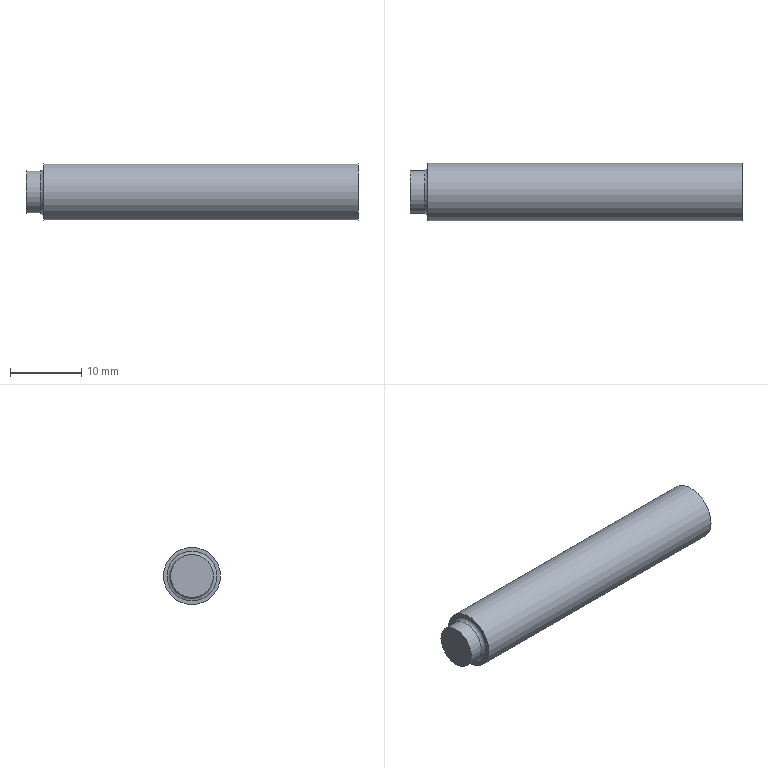Component | NX | PISTON_STRAIGHT_ROD | 1 solid | 8 faces | box 46.5 x 8 x 8 mm | volume 2097 mm3 | plane 4 | cylinder 3 | torus 1 | commonest cylinder face diameters 8 x1 6 x1 5 x1
STEP:
#1=CARTESIAN_POINT('',(0.,0.,0.));
#2=DIRECTION('',(0.,0.,1.));
#3=DIRECTION('',(1.,0.,0.));
#4=AXIS2_PLACEMENT_3D('',#1,#2,#3);
#5=CARTESIAN_POINT('',(-61.662,-53.5,38.5));
#6=VERTEX_POINT('',#5);
#7=CARTESIAN_POINT('',(-61.662,-50.,38.5));
#8=DIRECTION('',(1.,0.,0.));
#9=DIRECTION('',(0.,-1.,0.));
#10=AXIS2_PLACEMENT_3D('',#7,#8,#9);
#11=CIRCLE('',#10,3.5);
#12=CARTESIAN_POINT('',(-61.662,-50.,38.5));
#13=DIRECTION('',(-1.,0.,0.));
#14=DIRECTION('',(0.,-1.,0.));
#15=AXIS2_PLACEMENT_3D('',#12,#13,#14);
#16=PLANE('',#15);
#17=CARTESIAN_POINT('',(3.5,0.));
#18=CARTESIAN_POINT('',(3.5,-6.062));
#19=CARTESIAN_POINT('',(-1.75,-3.031));
#20=CARTESIAN_POINT('',(-7.,-0.));
#21=CARTESIAN_POINT('',(-1.75,3.031));
#22=CARTESIAN_POINT('',(3.5,6.062));
#23=CARTESIAN_POINT('',(3.5,0.));
#24=(BOUNDED_CURVE()B_SPLINE_CURVE(2,(#17,#18,#19,#20,#21,#22,#23),.UNSPECIFIED.,.T.,.F.)B_SPLINE_CURVE_WITH_KNOTS((1,2,2,2,2,1),(-2.094,0.,2.094,4.189,6.283,8.378),.UNSPECIFIED.)CURVE()GEOMETRIC_REPRESENTATION_ITEM()RATIONAL_B_SPLINE_CURVE((1.,0.5,1.,0.5,1.,0.5,1.))REPRESENTATION_ITEM(''));
#25=(GEOMETRIC_REPRESENTATION_CONTEXT(2)PARAMETRIC_REPRESENTATION_CONTEXT()REPRESENTATION_CONTEXT('',''));
#26=DEFINITIONAL_REPRESENTATION('',(#24),#25);
#27=PCURVE('',#16,#26);
#28=CARTESIAN_POINT('',(-62.162,-50.,38.5));
#29=DIRECTION('',(-1.,0.,0.));
#30=DIRECTION('',(0.,-1.,0.));
#31=AXIS2_PLACEMENT_3D('',#28,#29,#30);
#32=TOROIDAL_SURFACE('',#31,3.5,0.5);
#33=CARTESIAN_POINT('',(6.283,4.712));
#34=DIRECTION('',(-1.,0.));
#35=VECTOR('',#34,1.);
#36=LINE('',#33,#35);
#37=(GEOMETRIC_REPRESENTATION_CONTEXT(2)PARAMETRIC_REPRESENTATION_CONTEXT()REPRESENTATION_CONTEXT('',''));
#38=DEFINITIONAL_REPRESENTATION('',(#36),#37);
#39=PCURVE('',#32,#38);
#40=SURFACE_CURVE('',#11,(#27,#39),.PCURVE_S1.);
#41=EDGE_CURVE('',#6,#6,#40,.T.);
#42=ORIENTED_EDGE('',*,*,#41,.T.);
#43=EDGE_LOOP('',(#42));
#44=FACE_BOUND('',#43,.T.);
#45=CARTESIAN_POINT('',(-61.662,-54.,38.5));
#46=VERTEX_POINT('',#45);
#47=CARTESIAN_POINT('',(-61.662,-50.,38.5));
#48=DIRECTION('',(1.,0.,0.));
#49=DIRECTION('',(0.,-1.,0.));
#50=AXIS2_PLACEMENT_3D('',#47,#48,#49);
#51=CIRCLE('',#50,4.);
#52=CARTESIAN_POINT('',(4.,0.));
#53=CARTESIAN_POINT('',(4.,-6.928));
#54=CARTESIAN_POINT('',(-2.,-3.464));
#55=CARTESIAN_POINT('',(-8.,-0.));
#56=CARTESIAN_POINT('',(-2.,3.464));
#57=CARTESIAN_POINT('',(4.,6.928));
#58=CARTESIAN_POINT('',(4.,0.));
#59=(BOUNDED_CURVE()B_SPLINE_CURVE(2,(#52,#53,#54,#55,#56,#57,#58),.UNSPECIFIED.,.T.,.F.)B_SPLINE_CURVE_WITH_KNOTS((1,2,2,2,2,1),(-2.094,0.,2.094,4.189,6.283,8.378),.UNSPECIFIED.)CURVE()GEOMETRIC_REPRESENTATION_ITEM()RATIONAL_B_SPLINE_CURVE((1.,0.5,1.,0.5,1.,0.5,1.))REPRESENTATION_ITEM(''));
#60=(GEOMETRIC_REPRESENTATION_CONTEXT(2)PARAMETRIC_REPRESENTATION_CONTEXT()REPRESENTATION_CONTEXT('',''));
#61=DEFINITIONAL_REPRESENTATION('',(#59),#60);
#62=PCURVE('',#16,#61);
#63=CARTESIAN_POINT('',(-17.662,-50.,38.5));
#64=DIRECTION('',(-1.,0.,0.));
#65=DIRECTION('',(0.,-1.,0.));
#66=AXIS2_PLACEMENT_3D('',#63,#64,#65);
#67=CYLINDRICAL_SURFACE('',#66,4.);
#68=CARTESIAN_POINT('',(6.283,44.));
#69=DIRECTION('',(-1.,0.));
#70=VECTOR('',#69,1.);
#71=LINE('',#68,#70);
#72=(GEOMETRIC_REPRESENTATION_CONTEXT(2)PARAMETRIC_REPRESENTATION_CONTEXT()REPRESENTATION_CONTEXT('',''));
#73=DEFINITIONAL_REPRESENTATION('',(#71),#72);
#74=PCURVE('',#67,#73);
#75=SURFACE_CURVE('',#51,(#62,#74),.PCURVE_S1.);
#76=EDGE_CURVE('',#46,#46,#75,.T.);
#77=ORIENTED_EDGE('',*,*,#76,.F.);
#78=EDGE_LOOP('',(#77));
#79=FACE_BOUND('',#78,.T.);
#80=ADVANCED_FACE('',(#44,#79),#16,.T.);
#81=CARTESIAN_POINT('',(-17.662,-52.5,38.5));
#82=VERTEX_POINT('',#81);
#83=CARTESIAN_POINT('',(-17.662,-50.,38.5));
#84=DIRECTION('',(-1.,0.,0.));
#85=DIRECTION('',(0.,-1.,0.));
#86=AXIS2_PLACEMENT_3D('',#83,#84,#85);
#87=CIRCLE('',#86,2.5);
#88=CARTESIAN_POINT('',(-17.662,-50.,38.5));
#89=DIRECTION('',(1.,0.,0.));
#90=DIRECTION('',(0.,1.,0.));
#91=AXIS2_PLACEMENT_3D('',#88,#89,#90);
#92=PLANE('',#91);
#93=CARTESIAN_POINT('',(-2.5,0.));
#94=CARTESIAN_POINT('',(-2.5,4.33));
#95=CARTESIAN_POINT('',(1.25,2.165));
#96=CARTESIAN_POINT('',(5.,0.));
#97=CARTESIAN_POINT('',(1.25,-2.165));
#98=CARTESIAN_POINT('',(-2.5,-4.33));
#99=CARTESIAN_POINT('',(-2.5,0.));
#100=(BOUNDED_CURVE()B_SPLINE_CURVE(2,(#93,#94,#95,#96,#97,#98,#99),.UNSPECIFIED.,.T.,.F.)B_SPLINE_CURVE_WITH_KNOTS((1,2,2,2,2,1),(-2.094,0.,2.094,4.189,6.283,8.378),.UNSPECIFIED.)CURVE()GEOMETRIC_REPRESENTATION_ITEM()RATIONAL_B_SPLINE_CURVE((1.,0.5,1.,0.5,1.,0.5,1.))REPRESENTATION_ITEM(''));
#101=(GEOMETRIC_REPRESENTATION_CONTEXT(2)PARAMETRIC_REPRESENTATION_CONTEXT()REPRESENTATION_CONTEXT('',''));
#102=DEFINITIONAL_REPRESENTATION('',(#100),#101);
#103=PCURVE('',#92,#102);
#104=CARTESIAN_POINT('',(-27.162,-50.,38.5));
#105=DIRECTION('',(1.,0.,0.));
#106=DIRECTION('',(0.,1.,0.));
#107=AXIS2_PLACEMENT_3D('',#104,#105,#106);
#108=CYLINDRICAL_SURFACE('',#107,2.5);
#109=CARTESIAN_POINT('',(9.425,9.5));
#110=DIRECTION('',(-1.,0.));
#111=VECTOR('',#110,1.);
#112=LINE('',#109,#111);
#113=(GEOMETRIC_REPRESENTATION_CONTEXT(2)PARAMETRIC_REPRESENTATION_CONTEXT()REPRESENTATION_CONTEXT('',''));
#114=DEFINITIONAL_REPRESENTATION('',(#112),#113);
#115=PCURVE('',#108,#114);
#116=SURFACE_CURVE('',#87,(#103,#115),.PCURVE_S1.);
#117=EDGE_CURVE('',#82,#82,#116,.T.);
#118=ORIENTED_EDGE('',*,*,#117,.T.);
#119=EDGE_LOOP('',(#118));
#120=FACE_BOUND('',#119,.T.);
#121=CARTESIAN_POINT('',(-17.662,-54.,38.5));
#122=VERTEX_POINT('',#121);
#123=CARTESIAN_POINT('',(-17.662,-50.,38.5));
#124=DIRECTION('',(-1.,0.,0.));
#125=DIRECTION('',(0.,-1.,0.));
#126=AXIS2_PLACEMENT_3D('',#123,#124,#125);
#127=CIRCLE('',#126,4.);
#128=CARTESIAN_POINT('',(-4.,0.));
#129=CARTESIAN_POINT('',(-4.,6.928));
#130=CARTESIAN_POINT('',(2.,3.464));
#131=CARTESIAN_POINT('',(8.,0.));
#132=CARTESIAN_POINT('',(2.,-3.464));
#133=CARTESIAN_POINT('',(-4.,-6.928));
#134=CARTESIAN_POINT('',(-4.,0.));
#135=(BOUNDED_CURVE()B_SPLINE_CURVE(2,(#128,#129,#130,#131,#132,#133,#134),.UNSPECIFIED.,.T.,.F.)B_SPLINE_CURVE_WITH_KNOTS((1,2,2,2,2,1),(-2.094,0.,2.094,4.189,6.283,8.378),.UNSPECIFIED.)CURVE()GEOMETRIC_REPRESENTATION_ITEM()RATIONAL_B_SPLINE_CURVE((1.,0.5,1.,0.5,1.,0.5,1.))REPRESENTATION_ITEM(''));
#136=(GEOMETRIC_REPRESENTATION_CONTEXT(2)PARAMETRIC_REPRESENTATION_CONTEXT()REPRESENTATION_CONTEXT('',''));
#137=DEFINITIONAL_REPRESENTATION('',(#135),#136);
#138=PCURVE('',#92,#137);
#139=CARTESIAN_POINT('',(0.,0.));
#140=DIRECTION('',(1.,0.));
#141=VECTOR('',#140,1.);
#142=LINE('',#139,#141);
#143=(GEOMETRIC_REPRESENTATION_CONTEXT(2)PARAMETRIC_REPRESENTATION_CONTEXT()REPRESENTATION_CONTEXT('',''));
#144=DEFINITIONAL_REPRESENTATION('',(#142),#143);
#145=PCURVE('',#67,#144);
#146=SURFACE_CURVE('',#127,(#138,#145),.PCURVE_S1.);
#147=EDGE_CURVE('',#122,#122,#146,.T.);
#148=ORIENTED_EDGE('',*,*,#147,.F.);
#149=EDGE_LOOP('',(#148));
#150=FACE_BOUND('',#149,.T.);
#151=ADVANCED_FACE('',(#120,#150),#92,.T.);
#152=ORIENTED_EDGE('',*,*,#76,.T.);
#153=CARTESIAN_POINT('',(-17.662,-54.,38.5));
#154=CARTESIAN_POINT('',(-61.662,-54.,38.5));
#155=B_SPLINE_CURVE_WITH_KNOTS('',1,(#153,#154),.UNSPECIFIED.,.F.,.F.,(2,2),(0.,44.),.PIECEWISE_BEZIER_KNOTS.);
#156=CARTESIAN_POINT('',(0.,0.));
#157=DIRECTION('',(0.,1.));
#158=VECTOR('',#157,1.);
#159=LINE('',#156,#158);
#160=(GEOMETRIC_REPRESENTATION_CONTEXT(2)PARAMETRIC_REPRESENTATION_CONTEXT()REPRESENTATION_CONTEXT('',''));
#161=DEFINITIONAL_REPRESENTATION('',(#159),#160);
#162=PCURVE('',#67,#161);
#163=CARTESIAN_POINT('',(6.283,0.));
#164=DIRECTION('',(0.,1.));
#165=VECTOR('',#164,1.);
#166=LINE('',#163,#165);
#167=(GEOMETRIC_REPRESENTATION_CONTEXT(2)PARAMETRIC_REPRESENTATION_CONTEXT()REPRESENTATION_CONTEXT('',''));
#168=DEFINITIONAL_REPRESENTATION('',(#166),#167);
#169=PCURVE('',#67,#168);
#170=SEAM_CURVE('',#155,(#162,#169),.PCURVE_S1.);
#171=EDGE_CURVE('',#122,#46,#170,.T.);
#172=ORIENTED_EDGE('',*,*,#171,.F.);
#173=ORIENTED_EDGE('',*,*,#147,.T.);
#174=ORIENTED_EDGE('',*,*,#171,.T.);
#175=EDGE_LOOP('',(#152,#172,#173,#174));
#176=FACE_BOUND('',#175,.T.);
#177=ADVANCED_FACE('',(#176),#67,.T.);
#178=CARTESIAN_POINT('',(-64.162,-53.,38.5));
#179=VERTEX_POINT('',#178);
#180=CARTESIAN_POINT('',(-64.162,-50.,38.5));
#181=DIRECTION('',(-1.,0.,0.));
#182=DIRECTION('',(0.,-1.,0.));
#183=AXIS2_PLACEMENT_3D('',#180,#181,#182);
#184=CIRCLE('',#183,3.);
#185=CARTESIAN_POINT('',(-64.162,-50.,38.5));
#186=DIRECTION('',(-1.,0.,0.));
#187=DIRECTION('',(0.,-1.,0.));
#188=AXIS2_PLACEMENT_3D('',#185,#186,#187);
#189=PLANE('',#188);
#190=CARTESIAN_POINT('',(0.,0.));
#191=DIRECTION('',(1.,0.));
#192=AXIS2_PLACEMENT_2D('',#190,#191);
#193=CIRCLE('',#192,3.);
#194=(GEOMETRIC_REPRESENTATION_CONTEXT(2)PARAMETRIC_REPRESENTATION_CONTEXT()REPRESENTATION_CONTEXT('',''));
#195=DEFINITIONAL_REPRESENTATION('',(#193),#194);
#196=PCURVE('',#189,#195);
#197=CARTESIAN_POINT('',(-61.662,-50.,38.5));
#198=DIRECTION('',(-1.,0.,0.));
#199=DIRECTION('',(0.,-1.,0.));
#200=AXIS2_PLACEMENT_3D('',#197,#198,#199);
#201=CYLINDRICAL_SURFACE('',#200,3.);
#202=CARTESIAN_POINT('',(0.,2.5));
#203=DIRECTION('',(1.,0.));
#204=VECTOR('',#203,1.);
#205=LINE('',#202,#204);
#206=(GEOMETRIC_REPRESENTATION_CONTEXT(2)PARAMETRIC_REPRESENTATION_CONTEXT()REPRESENTATION_CONTEXT('',''));
#207=DEFINITIONAL_REPRESENTATION('',(#205),#206);
#208=PCURVE('',#201,#207);
#209=SURFACE_CURVE('',#184,(#196,#208),.PCURVE_S1.);
#210=EDGE_CURVE('',#179,#179,#209,.T.);
#211=ORIENTED_EDGE('',*,*,#210,.T.);
#212=EDGE_LOOP('',(#211));
#213=FACE_BOUND('',#212,.T.);
#214=ADVANCED_FACE('',(#213),#189,.T.);
#215=CARTESIAN_POINT('',(-62.162,-53.,38.5));
#216=VERTEX_POINT('',#215);
#217=CARTESIAN_POINT('',(-62.162,-50.,38.5));
#218=DIRECTION('',(-1.,0.,0.));
#219=DIRECTION('',(0.,-1.,0.));
#220=AXIS2_PLACEMENT_3D('',#217,#218,#219);
#221=CIRCLE('',#220,3.);
#222=CARTESIAN_POINT('',(0.,0.5));
#223=DIRECTION('',(1.,0.));
#224=VECTOR('',#223,1.);
#225=LINE('',#222,#224);
#226=(GEOMETRIC_REPRESENTATION_CONTEXT(2)PARAMETRIC_REPRESENTATION_CONTEXT()REPRESENTATION_CONTEXT('',''));
#227=DEFINITIONAL_REPRESENTATION('',(#225),#226);
#228=PCURVE('',#201,#227);
#229=CARTESIAN_POINT('',(0.,3.142));
#230=DIRECTION('',(1.,0.));
#231=VECTOR('',#230,1.);
#232=LINE('',#229,#231);
#233=(GEOMETRIC_REPRESENTATION_CONTEXT(2)PARAMETRIC_REPRESENTATION_CONTEXT()REPRESENTATION_CONTEXT('',''));
#234=DEFINITIONAL_REPRESENTATION('',(#232),#233);
#235=PCURVE('',#32,#234);
#236=SURFACE_CURVE('',#221,(#228,#235),.PCURVE_S1.);
#237=EDGE_CURVE('',#216,#216,#236,.T.);
#238=ORIENTED_EDGE('',*,*,#237,.T.);
#239=CARTESIAN_POINT('',(-62.162,-53.,38.5));
#240=CARTESIAN_POINT('',(-64.162,-53.,38.5));
#241=B_SPLINE_CURVE_WITH_KNOTS('',1,(#239,#240),.UNSPECIFIED.,.F.,.F.,(2,2),(0.5,2.5),.PIECEWISE_BEZIER_KNOTS.);
#242=CARTESIAN_POINT('',(6.283,0.));
#243=DIRECTION('',(0.,1.));
#244=VECTOR('',#243,1.);
#245=LINE('',#242,#244);
#246=(GEOMETRIC_REPRESENTATION_CONTEXT(2)PARAMETRIC_REPRESENTATION_CONTEXT()REPRESENTATION_CONTEXT('',''));
#247=DEFINITIONAL_REPRESENTATION('',(#245),#246);
#248=PCURVE('',#201,#247);
#249=CARTESIAN_POINT('',(0.,0.));
#250=DIRECTION('',(0.,1.));
#251=VECTOR('',#250,1.);
#252=LINE('',#249,#251);
#253=(GEOMETRIC_REPRESENTATION_CONTEXT(2)PARAMETRIC_REPRESENTATION_CONTEXT()REPRESENTATION_CONTEXT('',''));
#254=DEFINITIONAL_REPRESENTATION('',(#252),#253);
#255=PCURVE('',#201,#254);
#256=SEAM_CURVE('',#241,(#248,#255),.PCURVE_S1.);
#257=EDGE_CURVE('',#216,#179,#256,.T.);
#258=ORIENTED_EDGE('',*,*,#257,.T.);
#259=ORIENTED_EDGE('',*,*,#210,.F.);
#260=ORIENTED_EDGE('',*,*,#257,.F.);
#261=EDGE_LOOP('',(#238,#258,#259,#260));
#262=FACE_BOUND('',#261,.T.);
#263=ADVANCED_FACE('',(#262),#201,.T.);
#264=ORIENTED_EDGE('',*,*,#41,.T.);
#265=CARTESIAN_POINT('',(-62.162,-53.,38.5));
#266=CARTESIAN_POINT('',(-62.028,-53.,38.5));
#267=CARTESIAN_POINT('',(-61.898,-53.043,38.5));
#268=CARTESIAN_POINT('',(-61.786,-53.124,38.5));
#269=CARTESIAN_POINT('',(-61.704,-53.236,38.5));
#270=CARTESIAN_POINT('',(-61.662,-53.366,38.5));
#271=CARTESIAN_POINT('',(-61.662,-53.5,38.5));
#272=(BOUNDED_CURVE()B_SPLINE_CURVE(6,(#265,#266,#267,#268,#269,#270,#271),.UNSPECIFIED.,.F.,.F.)B_SPLINE_CURVE_WITH_KNOTS((7,7),(3.142,4.712),.PIECEWISE_BEZIER_KNOTS.)CURVE()GEOMETRIC_REPRESENTATION_ITEM()RATIONAL_B_SPLINE_CURVE((1.031,1.01,0.9979,0.994,0.9979,1.01,1.031))REPRESENTATION_ITEM(''));
#273=CARTESIAN_POINT('',(0.,0.));
#274=DIRECTION('',(0.,1.));
#275=VECTOR('',#274,1.);
#276=LINE('',#273,#275);
#277=(GEOMETRIC_REPRESENTATION_CONTEXT(2)PARAMETRIC_REPRESENTATION_CONTEXT()REPRESENTATION_CONTEXT('',''));
#278=DEFINITIONAL_REPRESENTATION('',(#276),#277);
#279=PCURVE('',#32,#278);
#280=CARTESIAN_POINT('',(6.283,0.));
#281=DIRECTION('',(0.,1.));
#282=VECTOR('',#281,1.);
#283=LINE('',#280,#282);
#284=(GEOMETRIC_REPRESENTATION_CONTEXT(2)PARAMETRIC_REPRESENTATION_CONTEXT()REPRESENTATION_CONTEXT('',''));
#285=DEFINITIONAL_REPRESENTATION('',(#283),#284);
#286=PCURVE('',#32,#285);
#287=SEAM_CURVE('',#272,(#279,#286),.PCURVE_S1.);
#288=EDGE_CURVE('',#216,#6,#287,.T.);
#289=ORIENTED_EDGE('',*,*,#288,.F.);
#290=ORIENTED_EDGE('',*,*,#237,.T.);
#291=ORIENTED_EDGE('',*,*,#288,.T.);
#292=EDGE_LOOP('',(#264,#289,#290,#291));
#293=FACE_BOUND('',#292,.F.);
#294=ADVANCED_FACE('',(#293),#32,.F.);
#295=CARTESIAN_POINT('',(-27.162,-52.5,38.5));
#296=VERTEX_POINT('',#295);
#297=CARTESIAN_POINT('',(-27.162,-50.,38.5));
#298=DIRECTION('',(1.,0.,0.));
#299=DIRECTION('',(0.,-1.,0.));
#300=AXIS2_PLACEMENT_3D('',#297,#298,#299);
#301=CIRCLE('',#300,2.5);
#302=CARTESIAN_POINT('',(3.142,0.));
#303=DIRECTION('',(1.,0.));
#304=VECTOR('',#303,1.);
#305=LINE('',#302,#304);
#306=(GEOMETRIC_REPRESENTATION_CONTEXT(2)PARAMETRIC_REPRESENTATION_CONTEXT()REPRESENTATION_CONTEXT('',''));
#307=DEFINITIONAL_REPRESENTATION('',(#305),#306);
#308=PCURVE('',#108,#307);
#309=CARTESIAN_POINT('',(-27.162,-50.,38.5));
#310=DIRECTION('',(-1.,0.,0.));
#311=DIRECTION('',(0.,-1.,0.));
#312=AXIS2_PLACEMENT_3D('',#309,#310,#311);
#313=PLANE('',#312);
#314=CARTESIAN_POINT('',(2.5,0.));
#315=CARTESIAN_POINT('',(2.5,-4.33));
#316=CARTESIAN_POINT('',(-1.25,-2.165));
#317=CARTESIAN_POINT('',(-5.,-0.));
#318=CARTESIAN_POINT('',(-1.25,2.165));
#319=CARTESIAN_POINT('',(2.5,4.33));
#320=CARTESIAN_POINT('',(2.5,0.));
#321=(BOUNDED_CURVE()B_SPLINE_CURVE(2,(#314,#315,#316,#317,#318,#319,#320),.UNSPECIFIED.,.T.,.F.)B_SPLINE_CURVE_WITH_KNOTS((1,2,2,2,2,1),(-2.094,0.,2.094,4.189,6.283,8.378),.UNSPECIFIED.)CURVE()GEOMETRIC_REPRESENTATION_ITEM()RATIONAL_B_SPLINE_CURVE((1.,0.5,1.,0.5,1.,0.5,1.))REPRESENTATION_ITEM(''));
#322=(GEOMETRIC_REPRESENTATION_CONTEXT(2)PARAMETRIC_REPRESENTATION_CONTEXT()REPRESENTATION_CONTEXT('',''));
#323=DEFINITIONAL_REPRESENTATION('',(#321),#322);
#324=PCURVE('',#313,#323);
#325=SURFACE_CURVE('',#301,(#308,#324),.PCURVE_S1.);
#326=EDGE_CURVE('',#296,#296,#325,.T.);
#327=ORIENTED_EDGE('',*,*,#326,.T.);
#328=CARTESIAN_POINT('',(-27.162,-52.5,38.5));
#329=CARTESIAN_POINT('',(-17.662,-52.5,38.5));
#330=B_SPLINE_CURVE_WITH_KNOTS('',1,(#328,#329),.UNSPECIFIED.,.F.,.F.,(2,2),(0.,9.5),.PIECEWISE_BEZIER_KNOTS.);
#331=CARTESIAN_POINT('',(9.425,0.));
#332=DIRECTION('',(0.,1.));
#333=VECTOR('',#332,1.);
#334=LINE('',#331,#333);
#335=(GEOMETRIC_REPRESENTATION_CONTEXT(2)PARAMETRIC_REPRESENTATION_CONTEXT()REPRESENTATION_CONTEXT('',''));
#336=DEFINITIONAL_REPRESENTATION('',(#334),#335);
#337=PCURVE('',#108,#336);
#338=CARTESIAN_POINT('',(3.142,0.));
#339=DIRECTION('',(0.,1.));
#340=VECTOR('',#339,1.);
#341=LINE('',#338,#340);
#342=(GEOMETRIC_REPRESENTATION_CONTEXT(2)PARAMETRIC_REPRESENTATION_CONTEXT()REPRESENTATION_CONTEXT('',''));
#343=DEFINITIONAL_REPRESENTATION('',(#341),#342);
#344=PCURVE('',#108,#343);
#345=SEAM_CURVE('',#330,(#337,#344),.PCURVE_S1.);
#346=EDGE_CURVE('',#296,#82,#345,.T.);
#347=ORIENTED_EDGE('',*,*,#346,.T.);
#348=ORIENTED_EDGE('',*,*,#117,.T.);
#349=ORIENTED_EDGE('',*,*,#346,.F.);
#350=EDGE_LOOP('',(#327,#347,#348,#349));
#351=FACE_BOUND('',#350,.F.);
#352=ADVANCED_FACE('',(#351),#108,.F.);
#353=ORIENTED_EDGE('',*,*,#326,.T.);
#354=EDGE_LOOP('',(#353));
#355=FACE_BOUND('',#354,.T.);
#356=ADVANCED_FACE('',(#355),#313,.F.);
#357=CLOSED_SHELL('',(#80,#151,#177,#214,#263,#294,#352,#356));
#358=MANIFOLD_SOLID_BREP('',#357);
#359=(LENGTH_UNIT()NAMED_UNIT(*)SI_UNIT(.MILLI.,.METRE.));
#360=UNCERTAINTY_MEASURE_WITH_UNIT(LENGTH_MEASURE(0.00001),#359,'','');
#361=(NAMED_UNIT(*)PLANE_ANGLE_UNIT()SI_UNIT($,.RADIAN.));
#362=(NAMED_UNIT(*)SI_UNIT($,.STERADIAN.)SOLID_ANGLE_UNIT());
#363=(GEOMETRIC_REPRESENTATION_CONTEXT(3)GLOBAL_UNCERTAINTY_ASSIGNED_CONTEXT((#360))GLOBAL_UNIT_ASSIGNED_CONTEXT((#359,#361,#362))REPRESENTATION_CONTEXT('',''));
#364=ADVANCED_BREP_SHAPE_REPRESENTATION('',(#4,#358),#363);